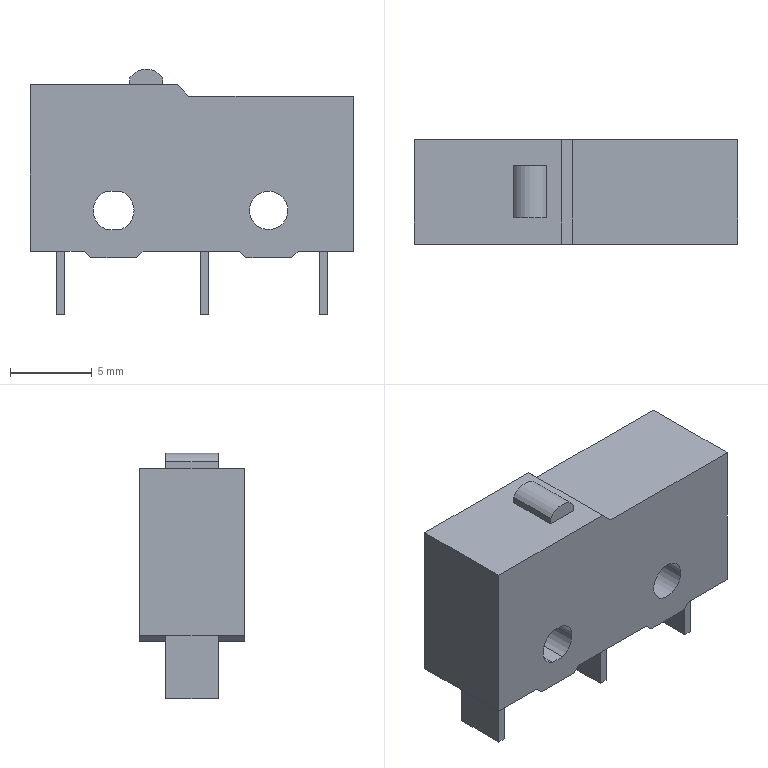Component | SolidWorks | SS_10GL2-1_SS_10GL2_BASE-1 | 1 solid | 43 faces | volume 1227 mm3 | plane 37 | cylinder 6 | commonest cylinder face diameters 2.5 x3 2.35 x2 2.4 x1